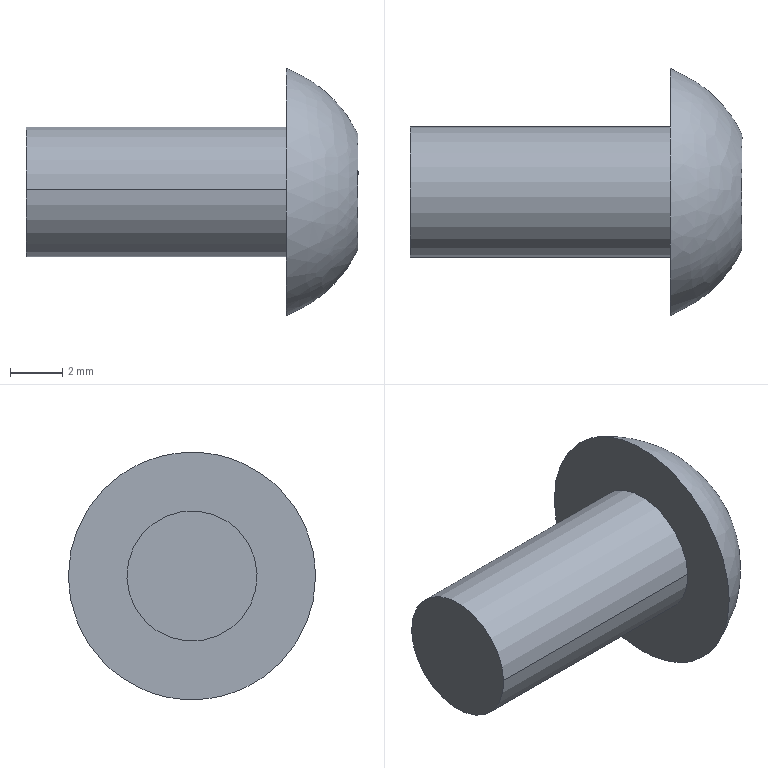Component | SolidWorks | ClampingAssembly-1_M5X10-1 | 1 solid | 18 faces | box 12.75 x 9.5 x 9.5 mm | volume 312 mm3 | plane 15 | cylinder 2 | spline 1 | commonest cylinder face diameters 5 x2 | material Standard Part
STEP:
#1=COLOUR_RGB('',0.7922,0.8196,0.9333);
#2=FILL_AREA_STYLE_COLOUR('',#1);
#3=FILL_AREA_STYLE('',(#2));
#4=SURFACE_STYLE_FILL_AREA(#3);
#5=SURFACE_SIDE_STYLE('',(#4));
#6=SURFACE_STYLE_USAGE(.BOTH.,#5);
#7=PRESENTATION_STYLE_ASSIGNMENT((#6));
#8=CARTESIAN_POINT('',(-1.203,2.698,-2.071));
#9=VERTEX_POINT('',#8);
#10=CARTESIAN_POINT('',(-1.203,2.501,-2.063));
#11=VERTEX_POINT('',#10);
#12=CARTESIAN_POINT('',(-1.203,2.6,-2.067));
#13=DIRECTION('',(1.,0.,-0.));
#14=DIRECTION('',(0.,0.9993,-0.03651));
#15=AXIS2_PLACEMENT_3D('',#12,#13,#14);
#16=CIRCLE('',#15,0.09843);
#17=EDGE_CURVE('',#9,#11,#16,.T.);
#18=ORIENTED_EDGE('',*,*,#17,.T.);
#19=CARTESIAN_POINT('',(-0.8091,2.501,-2.063));
#20=VERTEX_POINT('',#19);
#21=CARTESIAN_POINT('',(-1.203,2.501,-2.063));
#22=DIRECTION('',(1.,0.,-0.));
#23=VECTOR('',#22,39.37);
#24=LINE('',#21,#23);
#25=EDGE_CURVE('',#11,#20,#24,.T.);
#26=ORIENTED_EDGE('',*,*,#25,.T.);
#27=CARTESIAN_POINT('',(-0.8091,2.698,-2.071));
#28=VERTEX_POINT('',#27);
#29=CARTESIAN_POINT('',(-0.8091,2.6,-2.067));
#30=DIRECTION('',(-1.,-0.,0.));
#31=DIRECTION('',(0.,0.9993,-0.03651));
#32=AXIS2_PLACEMENT_3D('',#29,#30,#31);
#33=CIRCLE('',#32,0.09843);
#34=EDGE_CURVE('',#20,#28,#33,.T.);
#35=ORIENTED_EDGE('',*,*,#34,.T.);
#36=CARTESIAN_POINT('',(-1.203,2.698,-2.071));
#37=DIRECTION('',(1.,0.,-0.));
#38=VECTOR('',#37,39.37);
#39=LINE('',#36,#38);
#40=EDGE_CURVE('',#9,#28,#39,.T.);
#41=ORIENTED_EDGE('',*,*,#40,.F.);
#42=EDGE_LOOP('',(#18,#26,#35,#41));
#43=FACE_OUTER_BOUND('',#42,.T.);
#44=CARTESIAN_POINT('',(-1.203,2.6,-2.067));
#45=DIRECTION('',(1.,0.,-0.));
#46=DIRECTION('',(0.,0.9993,-0.03651));
#47=AXIS2_PLACEMENT_3D('',#44,#45,#46);
#48=CYLINDRICAL_SURFACE('',#47,0.09843);
#49=ADVANCED_FACE('',(#43),#48,.T.);
#50=ORIENTED_EDGE('',*,*,#25,.F.);
#51=CARTESIAN_POINT('',(-1.203,2.6,-2.067));
#52=DIRECTION('',(1.,0.,-0.));
#53=DIRECTION('',(0.,0.9993,-0.03651));
#54=AXIS2_PLACEMENT_3D('',#51,#52,#53);
#55=CIRCLE('',#54,0.09843);
#56=EDGE_CURVE('',#11,#9,#55,.T.);
#57=ORIENTED_EDGE('',*,*,#56,.T.);
#58=ORIENTED_EDGE('',*,*,#40,.T.);
#59=CARTESIAN_POINT('',(-0.8091,2.6,-2.067));
#60=DIRECTION('',(-1.,-0.,0.));
#61=DIRECTION('',(0.,0.9993,-0.03651));
#62=AXIS2_PLACEMENT_3D('',#59,#60,#61);
#63=CIRCLE('',#62,0.09843);
#64=EDGE_CURVE('',#28,#20,#63,.T.);
#65=ORIENTED_EDGE('',*,*,#64,.T.);
#66=EDGE_LOOP('',(#50,#57,#58,#65));
#67=FACE_OUTER_BOUND('',#66,.T.);
#68=CARTESIAN_POINT('',(-1.203,2.6,-2.067));
#69=DIRECTION('',(1.,0.,-0.));
#70=DIRECTION('',(0.,0.9993,-0.03651));
#71=AXIS2_PLACEMENT_3D('',#68,#69,#70);
#72=CYLINDRICAL_SURFACE('',#71,0.09843);
#73=ADVANCED_FACE('',(#67),#72,.T.);
#74=ORIENTED_EDGE('',*,*,#64,.F.);
#75=ORIENTED_EDGE('',*,*,#34,.F.);
#76=EDGE_LOOP('',(#74,#75));
#77=FACE_BOUND('',#76,.T.);
#78=CARTESIAN_POINT('',(-0.8091,2.607,-1.88));
#79=VERTEX_POINT('',#78);
#80=CARTESIAN_POINT('',(-0.8091,2.593,-2.254));
#81=VERTEX_POINT('',#80);
#82=CARTESIAN_POINT('',(-0.8091,2.607,-1.88));
#83=CARTESIAN_POINT('',(-0.8091,2.619,-1.88));
#84=CARTESIAN_POINT('',(-0.8091,2.631,-1.882));
#85=CARTESIAN_POINT('',(-0.8091,2.655,-1.888));
#86=CARTESIAN_POINT('',(-0.8091,2.667,-1.892));
#87=CARTESIAN_POINT('',(-0.8091,2.689,-1.902));
#88=CARTESIAN_POINT('',(-0.8091,2.699,-1.908));
#89=CARTESIAN_POINT('',(-0.8091,2.719,-1.922));
#90=CARTESIAN_POINT('',(-0.8091,2.729,-1.931));
#91=CARTESIAN_POINT('',(-0.8091,2.745,-1.949));
#92=CARTESIAN_POINT('',(-0.8091,2.753,-1.958));
#93=CARTESIAN_POINT('',(-0.8091,2.765,-1.979));
#94=CARTESIAN_POINT('',(-0.8091,2.771,-1.99));
#95=CARTESIAN_POINT('',(-0.8091,2.779,-2.013));
#96=CARTESIAN_POINT('',(-0.8091,2.782,-2.025));
#97=CARTESIAN_POINT('',(-0.8091,2.786,-2.049));
#98=CARTESIAN_POINT('',(-0.8091,2.787,-2.061));
#99=CARTESIAN_POINT('',(-0.8091,2.786,-2.086));
#100=CARTESIAN_POINT('',(-0.8091,2.785,-2.098));
#101=CARTESIAN_POINT('',(-0.8091,2.779,-2.122));
#102=CARTESIAN_POINT('',(-0.8091,2.775,-2.133));
#103=CARTESIAN_POINT('',(-0.8091,2.765,-2.156));
#104=CARTESIAN_POINT('',(-0.8091,2.759,-2.166));
#105=CARTESIAN_POINT('',(-0.8091,2.744,-2.186));
#106=CARTESIAN_POINT('',(-0.8091,2.736,-2.195));
#107=CARTESIAN_POINT('',(-0.8091,2.718,-2.212));
#108=CARTESIAN_POINT('',(-0.8091,2.708,-2.22));
#109=CARTESIAN_POINT('',(-0.8091,2.688,-2.232));
#110=CARTESIAN_POINT('',(-0.8091,2.677,-2.238));
#111=CARTESIAN_POINT('',(-0.8091,2.654,-2.246));
#112=CARTESIAN_POINT('',(-0.8091,2.642,-2.25));
#113=CARTESIAN_POINT('',(-0.8091,2.618,-2.253));
#114=CARTESIAN_POINT('',(-0.8091,2.605,-2.254));
#115=CARTESIAN_POINT('',(-0.8091,2.593,-2.254));
#116=B_SPLINE_CURVE_WITH_KNOTS('',3,(#82,#83,#84,#85,#86,#87,#88,#89,#90,#91,#92,#93,#94,#95,#96,#97,#98,#99,#100,#101,#102,#103,#104,#105,#106,#107,#108,#109,#110,#111,#112,#113,#114,#115),.UNSPECIFIED.,.F.,.F.,(4,2,2,2,2,2,2,2,2,2,2,2,2,2,2,2,4),(0.,0.000928,0.001856,0.002784,0.003712,0.00464,0.005568,0.006496,0.007424,0.008352,0.00928,0.01021,0.01114,0.01206,0.01299,0.01392,0.01485),.UNSPECIFIED.);
#117=EDGE_CURVE('',#79,#81,#116,.T.);
#118=ORIENTED_EDGE('',*,*,#117,.T.);
#119=CARTESIAN_POINT('',(-0.8091,2.593,-2.254));
#120=CARTESIAN_POINT('',(-0.8091,2.581,-2.253));
#121=CARTESIAN_POINT('',(-0.8091,2.569,-2.252));
#122=CARTESIAN_POINT('',(-0.8091,2.545,-2.246));
#123=CARTESIAN_POINT('',(-0.8091,2.533,-2.242));
#124=CARTESIAN_POINT('',(-0.8091,2.511,-2.232));
#125=CARTESIAN_POINT('',(-0.8091,2.5,-2.226));
#126=CARTESIAN_POINT('',(-0.8091,2.48,-2.211));
#127=CARTESIAN_POINT('',(-0.8091,2.471,-2.203));
#128=CARTESIAN_POINT('',(-0.8091,2.455,-2.185));
#129=CARTESIAN_POINT('',(-0.8091,2.447,-2.176));
#130=CARTESIAN_POINT('',(-0.8091,2.434,-2.155));
#131=CARTESIAN_POINT('',(-0.8091,2.429,-2.144));
#132=CARTESIAN_POINT('',(-0.8091,2.42,-2.121));
#133=CARTESIAN_POINT('',(-0.8091,2.417,-2.109));
#134=CARTESIAN_POINT('',(-0.8091,2.413,-2.085));
#135=CARTESIAN_POINT('',(-0.8091,2.413,-2.072));
#136=CARTESIAN_POINT('',(-0.8091,2.413,-2.048));
#137=CARTESIAN_POINT('',(-0.8091,2.415,-2.036));
#138=CARTESIAN_POINT('',(-0.8091,2.421,-2.012));
#139=CARTESIAN_POINT('',(-0.8091,2.425,-2.));
#140=CARTESIAN_POINT('',(-0.8091,2.435,-1.978));
#141=CARTESIAN_POINT('',(-0.8091,2.441,-1.967));
#142=CARTESIAN_POINT('',(-0.8091,2.455,-1.948));
#143=CARTESIAN_POINT('',(-0.8091,2.463,-1.938));
#144=CARTESIAN_POINT('',(-0.8091,2.481,-1.922));
#145=CARTESIAN_POINT('',(-0.8091,2.491,-1.914));
#146=CARTESIAN_POINT('',(-0.8091,2.512,-1.901));
#147=CARTESIAN_POINT('',(-0.8091,2.523,-1.896));
#148=CARTESIAN_POINT('',(-0.8091,2.546,-1.887));
#149=CARTESIAN_POINT('',(-0.8091,2.558,-1.884));
#150=CARTESIAN_POINT('',(-0.8091,2.582,-1.88));
#151=CARTESIAN_POINT('',(-0.8091,2.594,-1.88));
#152=CARTESIAN_POINT('',(-0.8091,2.607,-1.88));
#153=B_SPLINE_CURVE_WITH_KNOTS('',3,(#119,#120,#121,#122,#123,#124,#125,#126,#127,#128,#129,#130,#131,#132,#133,#134,#135,#136,#137,#138,#139,#140,#141,#142,#143,#144,#145,#146,#147,#148,#149,#150,#151,#152),.UNSPECIFIED.,.F.,.F.,(4,2,2,2,2,2,2,2,2,2,2,2,2,2,2,2,4),(0.01485,0.01578,0.0167,0.01763,0.01856,0.01949,0.02042,0.02134,0.02227,0.0232,0.02413,0.02506,0.02598,0.02691,0.02784,0.02877,0.0297),.UNSPECIFIED.);
#154=EDGE_CURVE('',#81,#79,#153,.T.);
#155=ORIENTED_EDGE('',*,*,#154,.T.);
#156=EDGE_LOOP('',(#118,#155));
#157=FACE_OUTER_BOUND('',#156,.T.);
#158=CARTESIAN_POINT('',(-0.8091,2.6,-2.067));
#159=DIRECTION('',(-1.,-0.,0.));
#160=DIRECTION('',(0.,-0.9993,0.03651));
#161=AXIS2_PLACEMENT_3D('',#158,#159,#160);
#162=PLANE('',#161);
#163=ADVANCED_FACE('',(#77,#157),#162,.T.);
#164=ORIENTED_EDGE('',*,*,#17,.F.);
#165=ORIENTED_EDGE('',*,*,#56,.F.);
#166=EDGE_LOOP('',(#164,#165));
#167=FACE_OUTER_BOUND('',#166,.T.);
#168=CARTESIAN_POINT('',(-1.203,2.6,-2.067));
#169=DIRECTION('',(-1.,-0.,0.));
#170=DIRECTION('',(0.,-0.9993,0.03651));
#171=AXIS2_PLACEMENT_3D('',#168,#169,#170);
#172=PLANE('',#171);
#173=ADVANCED_FACE('',(#167),#172,.T.);
#174=ORIENTED_EDGE('',*,*,#117,.F.);
#175=ORIENTED_EDGE('',*,*,#154,.F.);
#176=EDGE_LOOP('',(#174,#175));
#177=FACE_OUTER_BOUND('',#176,.T.);
#178=CARTESIAN_POINT('',(-0.7008,2.603,-1.98));
#179=VERTEX_POINT('',#178);
#180=CARTESIAN_POINT('',(-0.7008,2.597,-2.154));
#181=VERTEX_POINT('',#180);
#182=CARTESIAN_POINT('',(-0.7008,2.603,-1.98));
#183=CARTESIAN_POINT('',(-0.7008,2.609,-1.98));
#184=CARTESIAN_POINT('',(-0.7008,2.614,-1.981));
#185=CARTESIAN_POINT('',(-0.7008,2.626,-1.983));
#186=CARTESIAN_POINT('',(-0.7008,2.631,-1.985));
#187=CARTESIAN_POINT('',(-0.7008,2.641,-1.99));
#188=CARTESIAN_POINT('',(-0.7008,2.646,-1.993));
#189=CARTESIAN_POINT('',(-0.7008,2.656,-1.999));
#190=CARTESIAN_POINT('',(-0.7008,2.66,-2.003));
#191=CARTESIAN_POINT('',(-0.7008,2.672,-2.016));
#192=CARTESIAN_POINT('',(-0.7008,2.678,-2.026));
#193=CARTESIAN_POINT('',(-0.7008,2.686,-2.047));
#194=CARTESIAN_POINT('',(-0.7008,2.688,-2.059));
#195=CARTESIAN_POINT('',(-0.7008,2.687,-2.076));
#196=CARTESIAN_POINT('',(-0.7008,2.686,-2.082));
#197=CARTESIAN_POINT('',(-0.7008,2.684,-2.093));
#198=CARTESIAN_POINT('',(-0.7008,2.682,-2.098));
#199=CARTESIAN_POINT('',(-0.7008,2.677,-2.108));
#200=CARTESIAN_POINT('',(-0.7008,2.674,-2.113));
#201=CARTESIAN_POINT('',(-0.7008,2.667,-2.123));
#202=CARTESIAN_POINT('',(-0.7008,2.664,-2.127));
#203=CARTESIAN_POINT('',(-0.7008,2.655,-2.135));
#204=CARTESIAN_POINT('',(-0.7008,2.651,-2.138));
#205=CARTESIAN_POINT('',(-0.7008,2.641,-2.144));
#206=CARTESIAN_POINT('',(-0.7008,2.636,-2.147));
#207=CARTESIAN_POINT('',(-0.7008,2.625,-2.151));
#208=CARTESIAN_POINT('',(-0.7008,2.619,-2.152));
#209=CARTESIAN_POINT('',(-0.7008,2.608,-2.154));
#210=CARTESIAN_POINT('',(-0.7008,2.602,-2.154));
#211=CARTESIAN_POINT('',(-0.7008,2.597,-2.154));
#212=B_SPLINE_CURVE_WITH_KNOTS('',3,(#182,#183,#184,#185,#186,#187,#188,#189,#190,#191,#192,#193,#194,#195,#196,#197,#198,#199,#200,#201,#202,#203,#204,#205,#206,#207,#208,#209,#210,#211),.UNSPECIFIED.,.F.,.F.,(4,2,2,2,2,2,2,2,2,2,2,2,2,2,4),(0.,0.0004337,0.0008674,0.001301,0.001735,0.002602,0.00347,0.003903,0.004337,0.004771,0.005204,0.005638,0.006072,0.006506,0.006939),.UNSPECIFIED.);
#213=EDGE_CURVE('',#179,#181,#212,.T.);
#214=ORIENTED_EDGE('',*,*,#213,.T.);
#215=CARTESIAN_POINT('',(-0.7008,2.597,-2.154));
#216=CARTESIAN_POINT('',(-0.7008,2.591,-2.154));
#217=CARTESIAN_POINT('',(-0.7008,2.585,-2.153));
#218=CARTESIAN_POINT('',(-0.7008,2.574,-2.151));
#219=CARTESIAN_POINT('',(-0.7008,2.569,-2.149));
#220=CARTESIAN_POINT('',(-0.7008,2.558,-2.144));
#221=CARTESIAN_POINT('',(-0.7008,2.553,-2.141));
#222=CARTESIAN_POINT('',(-0.7008,2.544,-2.134));
#223=CARTESIAN_POINT('',(-0.7008,2.54,-2.131));
#224=CARTESIAN_POINT('',(-0.7008,2.528,-2.118));
#225=CARTESIAN_POINT('',(-0.7008,2.522,-2.108));
#226=CARTESIAN_POINT('',(-0.7008,2.514,-2.087));
#227=CARTESIAN_POINT('',(-0.7008,2.512,-2.075));
#228=CARTESIAN_POINT('',(-0.7008,2.513,-2.058));
#229=CARTESIAN_POINT('',(-0.7008,2.513,-2.052));
#230=CARTESIAN_POINT('',(-0.7008,2.516,-2.041));
#231=CARTESIAN_POINT('',(-0.7008,2.518,-2.036));
#232=CARTESIAN_POINT('',(-0.7008,2.523,-2.025));
#233=CARTESIAN_POINT('',(-0.7008,2.526,-2.02));
#234=CARTESIAN_POINT('',(-0.7008,2.532,-2.011));
#235=CARTESIAN_POINT('',(-0.7008,2.536,-2.007));
#236=CARTESIAN_POINT('',(-0.7008,2.545,-1.999));
#237=CARTESIAN_POINT('',(-0.7008,2.549,-1.996));
#238=CARTESIAN_POINT('',(-0.7008,2.559,-1.99));
#239=CARTESIAN_POINT('',(-0.7008,2.564,-1.987));
#240=CARTESIAN_POINT('',(-0.7008,2.575,-1.983));
#241=CARTESIAN_POINT('',(-0.7008,2.58,-1.982));
#242=CARTESIAN_POINT('',(-0.7008,2.591,-1.98));
#243=CARTESIAN_POINT('',(-0.7008,2.597,-1.979));
#244=CARTESIAN_POINT('',(-0.7008,2.603,-1.98));
#245=B_SPLINE_CURVE_WITH_KNOTS('',3,(#215,#216,#217,#218,#219,#220,#221,#222,#223,#224,#225,#226,#227,#228,#229,#230,#231,#232,#233,#234,#235,#236,#237,#238,#239,#240,#241,#242,#243,#244),.UNSPECIFIED.,.F.,.F.,(4,2,2,2,2,2,2,2,2,2,2,2,2,2,4),(0.006939,0.007373,0.007807,0.00824,0.008674,0.009542,0.01041,0.01084,0.01128,0.01171,0.01214,0.01258,0.01301,0.01344,0.01388),.UNSPECIFIED.);
#246=EDGE_CURVE('',#181,#179,#245,.T.);
#247=ORIENTED_EDGE('',*,*,#246,.T.);
#248=EDGE_LOOP('',(#214,#247));
#249=FACE_BOUND('',#248,.T.);
#250=CARTESIAN_POINT('',(-0.8573,2.542,-1.877));
#251=CARTESIAN_POINT('',(-0.7848,2.568,-1.878));
#252=CARTESIAN_POINT('',(-0.7848,2.645,-1.88));
#253=CARTESIAN_POINT('',(-0.8573,2.672,-1.881));
#254=CARTESIAN_POINT('',(-0.7855,2.343,-1.946));
#255=CARTESIAN_POINT('',(-0.4954,2.449,-1.95));
#256=CARTESIAN_POINT('',(-0.4954,2.758,-1.962));
#257=CARTESIAN_POINT('',(-0.7855,2.865,-1.965));
#258=CARTESIAN_POINT('',(-0.7855,2.335,-2.168));
#259=CARTESIAN_POINT('',(-0.4954,2.441,-2.172));
#260=CARTESIAN_POINT('',(-0.4954,2.75,-2.184));
#261=CARTESIAN_POINT('',(-0.7855,2.856,-2.187));
#262=CARTESIAN_POINT('',(-0.8573,2.528,-2.252));
#263=CARTESIAN_POINT('',(-0.7848,2.554,-2.253));
#264=CARTESIAN_POINT('',(-0.7848,2.632,-2.256));
#265=CARTESIAN_POINT('',(-0.8573,2.658,-2.257));
#266=(BOUNDED_SURFACE()B_SPLINE_SURFACE(3,3,((#250,#251,#252,#253),(#254,#255,#256,#257),(#258,#259,#260,#261),(#262,#263,#264,#265)),.UNSPECIFIED.,.F.,.F.,.T.)B_SPLINE_SURFACE_WITH_KNOTS((4,4),(4,4),(0.,1.),(0.,1.),.UNSPECIFIED.)GEOMETRIC_REPRESENTATION_ITEM()RATIONAL_B_SPLINE_SURFACE(((1.,0.5628,0.5628,1.),(0.5641,0.3175,0.3175,0.5641),(0.5641,0.3175,0.3175,0.5641),(1.,0.5628,0.5628,1.)))REPRESENTATION_ITEM('')SURFACE());
#267=ADVANCED_FACE('',(#177,#249),#266,.T.);
#268=CARTESIAN_POINT('',(-0.7008,2.568,-2.007));
#269=VERTEX_POINT('',#268);
#270=CARTESIAN_POINT('',(-0.7008,2.532,-2.064));
#271=VERTEX_POINT('',#270);
#272=CARTESIAN_POINT('',(-0.7008,2.568,-2.007));
#273=DIRECTION('',(0.,-0.5313,-0.8472));
#274=VECTOR('',#273,39.37);
#275=LINE('',#272,#274);
#276=EDGE_CURVE('',#269,#271,#275,.T.);
#277=ORIENTED_EDGE('',*,*,#276,.F.);
#278=CARTESIAN_POINT('',(-0.7008,2.636,-2.009));
#279=VERTEX_POINT('',#278);
#280=CARTESIAN_POINT('',(-0.7008,2.602,-2.008));
#281=DIRECTION('',(0.,-0.9993,0.03651));
#282=VECTOR('',#281,39.37);
#283=LINE('',#280,#282);
#284=EDGE_CURVE('',#279,#269,#283,.T.);
#285=ORIENTED_EDGE('',*,*,#284,.F.);
#286=CARTESIAN_POINT('',(-0.7008,2.668,-2.069));
#287=VERTEX_POINT('',#286);
#288=CARTESIAN_POINT('',(-0.7008,2.668,-2.069));
#289=DIRECTION('',(0.,-0.468,0.8837));
#290=VECTOR('',#289,39.37);
#291=LINE('',#288,#290);
#292=EDGE_CURVE('',#287,#279,#291,.T.);
#293=ORIENTED_EDGE('',*,*,#292,.F.);
#294=CARTESIAN_POINT('',(-0.7008,2.632,-2.127));
#295=VERTEX_POINT('',#294);
#296=CARTESIAN_POINT('',(-0.7008,2.632,-2.127));
#297=DIRECTION('',(-0.,0.5313,0.8472));
#298=VECTOR('',#297,39.37);
#299=LINE('',#296,#298);
#300=EDGE_CURVE('',#295,#287,#299,.T.);
#301=ORIENTED_EDGE('',*,*,#300,.F.);
#302=CARTESIAN_POINT('',(-0.7008,2.564,-2.125));
#303=VERTEX_POINT('',#302);
#304=CARTESIAN_POINT('',(-0.7008,2.598,-2.126));
#305=DIRECTION('',(-0.,0.9993,-0.03651));
#306=VECTOR('',#305,39.37);
#307=LINE('',#304,#306);
#308=EDGE_CURVE('',#303,#295,#307,.T.);
#309=ORIENTED_EDGE('',*,*,#308,.F.);
#310=CARTESIAN_POINT('',(-0.7008,2.532,-2.064));
#311=DIRECTION('',(-0.,0.468,-0.8837));
#312=VECTOR('',#311,39.37);
#313=LINE('',#310,#312);
#314=EDGE_CURVE('',#271,#303,#313,.T.);
#315=ORIENTED_EDGE('',*,*,#314,.F.);
#316=EDGE_LOOP('',(#277,#285,#293,#301,#309,#315));
#317=FACE_BOUND('',#316,.T.);
#318=ORIENTED_EDGE('',*,*,#213,.F.);
#319=ORIENTED_EDGE('',*,*,#246,.F.);
#320=EDGE_LOOP('',(#318,#319));
#321=FACE_OUTER_BOUND('',#320,.T.);
#322=CARTESIAN_POINT('',(-0.7008,2.6,-2.067));
#323=DIRECTION('',(-1.,-0.,0.));
#324=DIRECTION('',(0.,-0.9993,0.03651));
#325=AXIS2_PLACEMENT_3D('',#322,#323,#324);
#326=PLANE('',#325);
#327=ADVANCED_FACE('',(#317,#321),#326,.F.);
#328=CARTESIAN_POINT('',(-0.7622,2.564,-2.125));
#329=VERTEX_POINT('',#328);
#330=CARTESIAN_POINT('',(-0.7622,2.532,-2.064));
#331=VERTEX_POINT('',#330);
#332=CARTESIAN_POINT('',(-0.7622,2.564,-2.125));
#333=DIRECTION('',(0.,-0.468,0.8837));
#334=VECTOR('',#333,39.37);
#335=LINE('',#332,#334);
#336=EDGE_CURVE('',#329,#331,#335,.T.);
#337=ORIENTED_EDGE('',*,*,#336,.T.);
#338=CARTESIAN_POINT('',(-0.7622,2.532,-2.064));
#339=DIRECTION('',(1.,0.,-0.));
#340=VECTOR('',#339,39.37);
#341=LINE('',#338,#340);
#342=EDGE_CURVE('',#331,#271,#341,.T.);
#343=ORIENTED_EDGE('',*,*,#342,.T.);
#344=ORIENTED_EDGE('',*,*,#314,.T.);
#345=CARTESIAN_POINT('',(-0.7622,2.564,-2.125));
#346=DIRECTION('',(-1.,-0.,0.));
#347=VECTOR('',#346,39.37);
#348=LINE('',#345,#347);
#349=EDGE_CURVE('',#303,#329,#348,.T.);
#350=ORIENTED_EDGE('',*,*,#349,.T.);
#351=EDGE_LOOP('',(#337,#343,#344,#350));
#352=FACE_OUTER_BOUND('',#351,.T.);
#353=CARTESIAN_POINT('',(-0.7622,2.564,-2.125));
#354=DIRECTION('',(-0.,0.8837,0.468));
#355=DIRECTION('',(-0.,0.468,-0.8837));
#356=AXIS2_PLACEMENT_3D('',#353,#354,#355);
#357=PLANE('',#356);
#358=ADVANCED_FACE('',(#352),#357,.T.);
#359=CARTESIAN_POINT('',(-0.7622,2.568,-2.007));
#360=VERTEX_POINT('',#359);
#361=CARTESIAN_POINT('',(-0.7622,2.532,-2.064));
#362=DIRECTION('',(-0.,0.5313,0.8472));
#363=VECTOR('',#362,39.37);
#364=LINE('',#361,#363);
#365=EDGE_CURVE('',#331,#360,#364,.T.);
#366=ORIENTED_EDGE('',*,*,#365,.T.);
#367=CARTESIAN_POINT('',(-0.7622,2.568,-2.007));
#368=DIRECTION('',(1.,0.,-0.));
#369=VECTOR('',#368,39.37);
#370=LINE('',#367,#369);
#371=EDGE_CURVE('',#360,#269,#370,.T.);
#372=ORIENTED_EDGE('',*,*,#371,.T.);
#373=ORIENTED_EDGE('',*,*,#276,.T.);
#374=ORIENTED_EDGE('',*,*,#342,.F.);
#375=EDGE_LOOP('',(#366,#372,#373,#374));
#376=FACE_OUTER_BOUND('',#375,.T.);
#377=CARTESIAN_POINT('',(-0.7622,2.532,-2.064));
#378=DIRECTION('',(-0.,0.8472,-0.5313));
#379=DIRECTION('',(0.,-0.5313,-0.8472));
#380=AXIS2_PLACEMENT_3D('',#377,#378,#379);
#381=PLANE('',#380);
#382=ADVANCED_FACE('',(#376),#381,.T.);
#383=CARTESIAN_POINT('',(-0.7622,2.636,-2.009));
#384=VERTEX_POINT('',#383);
#385=CARTESIAN_POINT('',(-0.7622,2.568,-2.007));
#386=DIRECTION('',(-0.,0.9993,-0.03651));
#387=VECTOR('',#386,39.37);
#388=LINE('',#385,#387);
#389=EDGE_CURVE('',#360,#384,#388,.T.);
#390=ORIENTED_EDGE('',*,*,#389,.T.);
#391=CARTESIAN_POINT('',(-0.7622,2.636,-2.009));
#392=DIRECTION('',(1.,0.,-0.));
#393=VECTOR('',#392,39.37);
#394=LINE('',#391,#393);
#395=EDGE_CURVE('',#384,#279,#394,.T.);
#396=ORIENTED_EDGE('',*,*,#395,.T.);
#397=ORIENTED_EDGE('',*,*,#284,.T.);
#398=ORIENTED_EDGE('',*,*,#371,.F.);
#399=EDGE_LOOP('',(#390,#396,#397,#398));
#400=FACE_OUTER_BOUND('',#399,.T.);
#401=CARTESIAN_POINT('',(-0.7622,2.568,-2.007));
#402=DIRECTION('',(-0.,-0.03651,-0.9993));
#403=DIRECTION('',(0.,-0.9993,0.03651));
#404=AXIS2_PLACEMENT_3D('',#401,#402,#403);
#405=PLANE('',#404);
#406=ADVANCED_FACE('',(#400),#405,.T.);
#407=CARTESIAN_POINT('',(-0.7622,2.668,-2.069));
#408=VERTEX_POINT('',#407);
#409=CARTESIAN_POINT('',(-0.7622,2.636,-2.009));
#410=DIRECTION('',(-0.,0.468,-0.8837));
#411=VECTOR('',#410,39.37);
#412=LINE('',#409,#411);
#413=EDGE_CURVE('',#384,#408,#412,.T.);
#414=ORIENTED_EDGE('',*,*,#413,.T.);
#415=CARTESIAN_POINT('',(-0.7622,2.668,-2.069));
#416=DIRECTION('',(1.,0.,-0.));
#417=VECTOR('',#416,39.37);
#418=LINE('',#415,#417);
#419=EDGE_CURVE('',#408,#287,#418,.T.);
#420=ORIENTED_EDGE('',*,*,#419,.T.);
#421=ORIENTED_EDGE('',*,*,#292,.T.);
#422=ORIENTED_EDGE('',*,*,#395,.F.);
#423=EDGE_LOOP('',(#414,#420,#421,#422));
#424=FACE_OUTER_BOUND('',#423,.T.);
#425=CARTESIAN_POINT('',(-0.7622,2.636,-2.009));
#426=DIRECTION('',(0.,-0.8837,-0.468));
#427=DIRECTION('',(0.,-0.468,0.8837));
#428=AXIS2_PLACEMENT_3D('',#425,#426,#427);
#429=PLANE('',#428);
#430=ADVANCED_FACE('',(#424),#429,.T.);
#431=CARTESIAN_POINT('',(-0.7622,2.632,-2.127));
#432=VERTEX_POINT('',#431);
#433=CARTESIAN_POINT('',(-0.7622,2.668,-2.069));
#434=DIRECTION('',(0.,-0.5313,-0.8472));
#435=VECTOR('',#434,39.37);
#436=LINE('',#433,#435);
#437=EDGE_CURVE('',#408,#432,#436,.T.);
#438=ORIENTED_EDGE('',*,*,#437,.T.);
#439=CARTESIAN_POINT('',(-0.7622,2.632,-2.127));
#440=DIRECTION('',(1.,0.,-0.));
#441=VECTOR('',#440,39.37);
#442=LINE('',#439,#441);
#443=EDGE_CURVE('',#432,#295,#442,.T.);
#444=ORIENTED_EDGE('',*,*,#443,.T.);
#445=ORIENTED_EDGE('',*,*,#300,.T.);
#446=ORIENTED_EDGE('',*,*,#419,.F.);
#447=EDGE_LOOP('',(#438,#444,#445,#446));
#448=FACE_OUTER_BOUND('',#447,.T.);
#449=CARTESIAN_POINT('',(-0.7622,2.668,-2.069));
#450=DIRECTION('',(0.,-0.8472,0.5313));
#451=DIRECTION('',(-0.,0.5313,0.8472));
#452=AXIS2_PLACEMENT_3D('',#449,#450,#451);
#453=PLANE('',#452);
#454=ADVANCED_FACE('',(#448),#453,.T.);
#455=CARTESIAN_POINT('',(-0.7622,2.632,-2.127));
#456=DIRECTION('',(0.,-0.9993,0.03651));
#457=VECTOR('',#456,39.37);
#458=LINE('',#455,#457);
#459=EDGE_CURVE('',#432,#329,#458,.T.);
#460=ORIENTED_EDGE('',*,*,#459,.T.);
#461=ORIENTED_EDGE('',*,*,#349,.F.);
#462=ORIENTED_EDGE('',*,*,#308,.T.);
#463=ORIENTED_EDGE('',*,*,#443,.F.);
#464=EDGE_LOOP('',(#460,#461,#462,#463));
#465=FACE_OUTER_BOUND('',#464,.T.);
#466=CARTESIAN_POINT('',(-0.7622,2.632,-2.127));
#467=DIRECTION('',(0.,0.03651,0.9993));
#468=DIRECTION('',(-0.,0.9993,-0.03651));
#469=AXIS2_PLACEMENT_3D('',#466,#467,#468);
#470=PLANE('',#469);
#471=ADVANCED_FACE('',(#465),#470,.T.);
#472=CARTESIAN_POINT('',(-0.7963,2.6,-2.067));
#473=VERTEX_POINT('',#472);
#474=CARTESIAN_POINT('',(-0.7963,2.6,-2.067));
#475=DIRECTION('',(0.4472,-0.4752,-0.7578));
#476=VECTOR('',#475,39.37);
#477=LINE('',#474,#476);
#478=EDGE_CURVE('',#473,#329,#477,.T.);
#479=ORIENTED_EDGE('',*,*,#478,.F.);
#480=CARTESIAN_POINT('',(-0.7759,2.559,-2.065));
#481=DIRECTION('',(-0.4472,0.8938,-0.03265));
#482=VECTOR('',#481,39.37);
#483=LINE('',#480,#482);
#484=EDGE_CURVE('',#331,#473,#483,.T.);
#485=ORIENTED_EDGE('',*,*,#484,.F.);
#486=ORIENTED_EDGE('',*,*,#336,.F.);
#487=EDGE_LOOP('',(#479,#485,#486));
#488=FACE_OUTER_BOUND('',#487,.T.);
#489=CARTESIAN_POINT('',(-0.7622,2.564,-2.125));
#490=DIRECTION('',(-0.866,-0.4419,-0.234));
#491=DIRECTION('',(0.4472,-0.8938,0.03265));
#492=AXIS2_PLACEMENT_3D('',#489,#490,#491);
#493=PLANE('',#492);
#494=ADVANCED_FACE('',(#488),#493,.F.);
#495=CARTESIAN_POINT('',(-0.7963,2.6,-2.067));
#496=DIRECTION('',(0.4472,0.4186,-0.7904));
#497=VECTOR('',#496,39.37);
#498=LINE('',#495,#497);
#499=EDGE_CURVE('',#473,#432,#498,.T.);
#500=ORIENTED_EDGE('',*,*,#499,.F.);
#501=ORIENTED_EDGE('',*,*,#478,.T.);
#502=ORIENTED_EDGE('',*,*,#459,.F.);
#503=EDGE_LOOP('',(#500,#501,#502));
#504=FACE_OUTER_BOUND('',#503,.T.);
#505=CARTESIAN_POINT('',(-0.7622,2.632,-2.127));
#506=DIRECTION('',(-0.866,-0.01825,-0.4997));
#507=DIRECTION('',(-0.5,0.03162,0.8654));
#508=AXIS2_PLACEMENT_3D('',#505,#506,#507);
#509=PLANE('',#508);
#510=ADVANCED_FACE('',(#504),#509,.F.);
#511=ORIENTED_EDGE('',*,*,#484,.T.);
#512=CARTESIAN_POINT('',(-0.7622,2.568,-2.007));
#513=DIRECTION('',(-0.4472,0.4186,-0.7904));
#514=VECTOR('',#513,39.37);
#515=LINE('',#512,#514);
#516=EDGE_CURVE('',#360,#473,#515,.T.);
#517=ORIENTED_EDGE('',*,*,#516,.F.);
#518=ORIENTED_EDGE('',*,*,#365,.F.);
#519=EDGE_LOOP('',(#511,#517,#518));
#520=FACE_OUTER_BOUND('',#519,.T.);
#521=CARTESIAN_POINT('',(-0.7622,2.532,-2.064));
#522=DIRECTION('',(-0.866,-0.4236,0.2656));
#523=DIRECTION('',(0.4472,-0.8938,0.03265));
#524=AXIS2_PLACEMENT_3D('',#521,#522,#523);
#525=PLANE('',#524);
#526=ADVANCED_FACE('',(#520),#525,.F.);
#527=CARTESIAN_POINT('',(-0.7622,2.668,-2.069));
#528=DIRECTION('',(0.4472,0.8938,-0.03265));
#529=VECTOR('',#528,39.37);
#530=LINE('',#527,#529);
#531=EDGE_CURVE('',#473,#408,#530,.T.);
#532=ORIENTED_EDGE('',*,*,#531,.F.);
#533=ORIENTED_EDGE('',*,*,#499,.T.);
#534=ORIENTED_EDGE('',*,*,#437,.F.);
#535=EDGE_LOOP('',(#532,#533,#534));
#536=FACE_OUTER_BOUND('',#535,.T.);
#537=CARTESIAN_POINT('',(-0.7622,2.668,-2.069));
#538=DIRECTION('',(-0.866,0.4236,-0.2656));
#539=DIRECTION('',(-0.4472,-0.8938,0.03265));
#540=AXIS2_PLACEMENT_3D('',#537,#538,#539);
#541=PLANE('',#540);
#542=ADVANCED_FACE('',(#536),#541,.F.);
#543=ORIENTED_EDGE('',*,*,#516,.T.);
#544=CARTESIAN_POINT('',(-0.7622,2.636,-2.009));
#545=DIRECTION('',(-0.4472,-0.4752,-0.7578));
#546=VECTOR('',#545,39.37);
#547=LINE('',#544,#546);
#548=EDGE_CURVE('',#384,#473,#547,.T.);
#549=ORIENTED_EDGE('',*,*,#548,.F.);
#550=ORIENTED_EDGE('',*,*,#389,.F.);
#551=EDGE_LOOP('',(#543,#549,#550));
#552=FACE_OUTER_BOUND('',#551,.T.);
#553=CARTESIAN_POINT('',(-0.7622,2.568,-2.007));
#554=DIRECTION('',(-0.866,0.01825,0.4997));
#555=DIRECTION('',(0.5,0.03162,0.8654));
#556=AXIS2_PLACEMENT_3D('',#553,#554,#555);
#557=PLANE('',#556);
#558=ADVANCED_FACE('',(#552),#557,.F.);
#559=ORIENTED_EDGE('',*,*,#548,.T.);
#560=ORIENTED_EDGE('',*,*,#531,.T.);
#561=ORIENTED_EDGE('',*,*,#413,.F.);
#562=EDGE_LOOP('',(#559,#560,#561));
#563=FACE_OUTER_BOUND('',#562,.T.);
#564=CARTESIAN_POINT('',(-0.7622,2.636,-2.009));
#565=DIRECTION('',(-0.866,0.4419,0.234));
#566=DIRECTION('',(-0.4472,-0.8938,0.03265));
#567=AXIS2_PLACEMENT_3D('',#564,#565,#566);
#568=PLANE('',#567);
#569=ADVANCED_FACE('',(#563),#568,.F.);
#570=CLOSED_SHELL('',(#49,#73,#163,#173,#267,#327,#358,#382,#406,#430,#454,#471,#494,#510,#526,#542,#558,#569));
#571=MANIFOLD_SOLID_BREP('',#570);
#572=STYLED_ITEM('',(#7),#571);
#573=(LENGTH_UNIT()NAMED_UNIT(*)SI_UNIT($,.METRE.));
#574=LENGTH_MEASURE_WITH_UNIT(LENGTH_MEASURE(0.0254),#573);
#575=DIMENSIONAL_EXPONENTS(1.,0.,0.,0.,0.,0.,0.);
#576=(CONVERSION_BASED_UNIT('',#574)LENGTH_UNIT()NAMED_UNIT(#575));
#577=UNCERTAINTY_MEASURE_WITH_UNIT(LENGTH_MEASURE(0.00001),#576,'','');
#578=(NAMED_UNIT(*)PLANE_ANGLE_UNIT()SI_UNIT($,.RADIAN.));
#579=(NAMED_UNIT(*)SI_UNIT($,.STERADIAN.)SOLID_ANGLE_UNIT());
#580=(GEOMETRIC_REPRESENTATION_CONTEXT(3)GLOBAL_UNCERTAINTY_ASSIGNED_CONTEXT((#577))GLOBAL_UNIT_ASSIGNED_CONTEXT((#576,#578,#579))REPRESENTATION_CONTEXT('',''));
#581=MECHANICAL_DESIGN_GEOMETRIC_PRESENTATION_REPRESENTATION('',(#572),#580);
#582=PRESENTATION_LAYER_ASSIGNMENT('','',(#572));
#583=CARTESIAN_POINT('',(0.,0.,0.));
#584=DIRECTION('',(0.,0.,1.));
#585=DIRECTION('',(1.,0.,0.));
#586=AXIS2_PLACEMENT_3D('',#583,#584,#585);
#587=(LENGTH_UNIT()NAMED_UNIT(*)SI_UNIT($,.METRE.));
#588=LENGTH_MEASURE_WITH_UNIT(LENGTH_MEASURE(0.0254),#587);
#589=DIMENSIONAL_EXPONENTS(1.,0.,0.,0.,0.,0.,0.);
#590=(CONVERSION_BASED_UNIT('',#588)LENGTH_UNIT()NAMED_UNIT(#589));
#591=UNCERTAINTY_MEASURE_WITH_UNIT(LENGTH_MEASURE(0.00001),#590,'','');
#592=(NAMED_UNIT(*)PLANE_ANGLE_UNIT()SI_UNIT($,.RADIAN.));
#593=(NAMED_UNIT(*)SI_UNIT($,.STERADIAN.)SOLID_ANGLE_UNIT());
#594=(GEOMETRIC_REPRESENTATION_CONTEXT(3)GLOBAL_UNCERTAINTY_ASSIGNED_CONTEXT((#591))GLOBAL_UNIT_ASSIGNED_CONTEXT((#590,#592,#593))REPRESENTATION_CONTEXT('',''));
#595=ADVANCED_BREP_SHAPE_REPRESENTATION('',(#571,#586),#594);